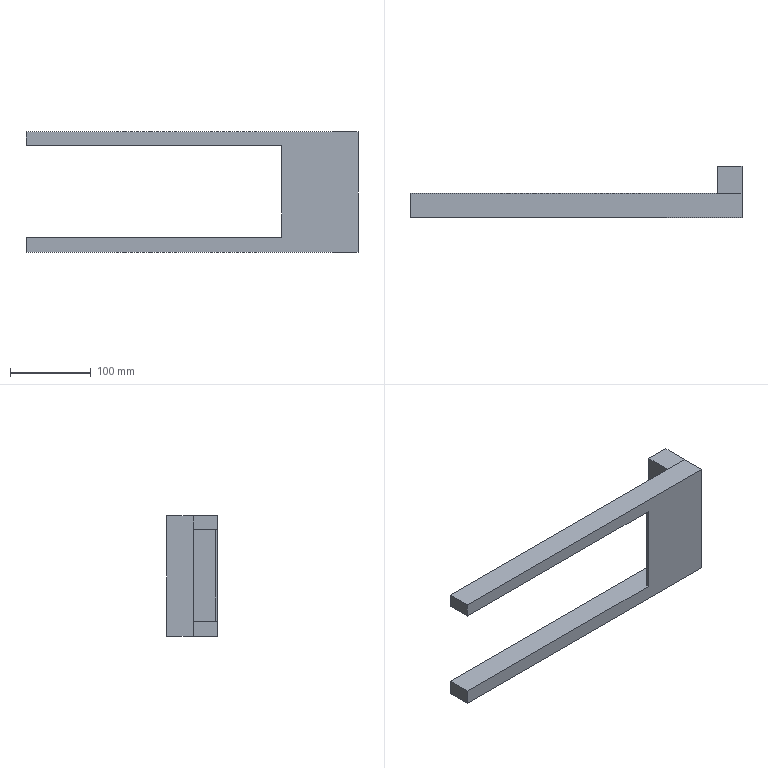Component | SolidWorks | w-1 | 2 solids | 18 faces | box 412.36 x 63.27 x 149.69 mm | volume 706312 mm3 | plane 18
STEP:
#1=CARTESIAN_POINT('',(5.039,-6.626,-2.108));
#2=VERTEX_POINT('',#1);
#3=CARTESIAN_POINT('',(5.039,-6.626,-2.842));
#4=VERTEX_POINT('',#3);
#5=CARTESIAN_POINT('',(5.039,-6.626,3.051));
#6=DIRECTION('',(0.,0.,-1.));
#7=VECTOR('',#6,39.37);
#8=LINE('',#5,#7);
#9=EDGE_CURVE('',#2,#4,#8,.T.);
#10=ORIENTED_EDGE('',*,*,#9,.F.);
#11=CARTESIAN_POINT('',(5.039,-5.445,-2.108));
#12=VERTEX_POINT('',#11);
#13=CARTESIAN_POINT('',(5.039,-8.83,-2.108));
#14=DIRECTION('',(0.,1.,0.));
#15=VECTOR('',#14,39.37);
#16=LINE('',#13,#15);
#17=EDGE_CURVE('',#2,#12,#16,.T.);
#18=ORIENTED_EDGE('',*,*,#17,.T.);
#19=CARTESIAN_POINT('',(5.039,-5.445,-2.842));
#20=VERTEX_POINT('',#19);
#21=CARTESIAN_POINT('',(5.039,-5.445,3.051));
#22=DIRECTION('',(0.,0.,-1.));
#23=VECTOR('',#22,39.37);
#24=LINE('',#21,#23);
#25=EDGE_CURVE('',#12,#20,#24,.T.);
#26=ORIENTED_EDGE('',*,*,#25,.T.);
#27=CARTESIAN_POINT('',(5.039,-6.626,-2.842));
#28=DIRECTION('',(0.,1.,0.));
#29=VECTOR('',#28,39.37);
#30=LINE('',#27,#29);
#31=EDGE_CURVE('',#4,#20,#30,.T.);
#32=ORIENTED_EDGE('',*,*,#31,.F.);
#33=EDGE_LOOP('',(#10,#18,#26,#32));
#34=FACE_OUTER_BOUND('',#33,.T.);
#35=CARTESIAN_POINT('',(5.039,-6.626,3.051));
#36=DIRECTION('',(1.,0.,0.));
#37=DIRECTION('',(0.,-1.,0.));
#38=AXIS2_PLACEMENT_3D('',#35,#36,#37);
#39=PLANE('',#38);
#40=ADVANCED_FACE('',(#34),#39,.F.);
#41=CARTESIAN_POINT('',(5.039,-5.445,3.051));
#42=VERTEX_POINT('',#41);
#43=CARTESIAN_POINT('',(5.039,-5.445,2.387));
#44=VERTEX_POINT('',#43);
#45=CARTESIAN_POINT('',(5.039,-5.445,3.051));
#46=DIRECTION('',(0.,0.,-1.));
#47=VECTOR('',#46,39.37);
#48=LINE('',#45,#47);
#49=EDGE_CURVE('',#42,#44,#48,.T.);
#50=ORIENTED_EDGE('',*,*,#49,.T.);
#51=CARTESIAN_POINT('',(5.039,-6.626,2.387));
#52=VERTEX_POINT('',#51);
#53=CARTESIAN_POINT('',(5.039,-8.83,2.387));
#54=DIRECTION('',(0.,1.,0.));
#55=VECTOR('',#54,39.37);
#56=LINE('',#53,#55);
#57=EDGE_CURVE('',#52,#44,#56,.T.);
#58=ORIENTED_EDGE('',*,*,#57,.F.);
#59=CARTESIAN_POINT('',(5.039,-6.626,3.051));
#60=VERTEX_POINT('',#59);
#61=CARTESIAN_POINT('',(5.039,-6.626,3.051));
#62=DIRECTION('',(0.,0.,-1.));
#63=VECTOR('',#62,39.37);
#64=LINE('',#61,#63);
#65=EDGE_CURVE('',#60,#52,#64,.T.);
#66=ORIENTED_EDGE('',*,*,#65,.F.);
#67=CARTESIAN_POINT('',(5.039,-6.626,3.051));
#68=DIRECTION('',(0.,1.,0.));
#69=VECTOR('',#68,39.37);
#70=LINE('',#67,#69);
#71=EDGE_CURVE('',#60,#42,#70,.T.);
#72=ORIENTED_EDGE('',*,*,#71,.T.);
#73=EDGE_LOOP('',(#50,#58,#66,#72));
#74=FACE_OUTER_BOUND('',#73,.T.);
#75=CARTESIAN_POINT('',(5.039,-6.626,3.051));
#76=DIRECTION('',(1.,0.,0.));
#77=DIRECTION('',(0.,-1.,0.));
#78=AXIS2_PLACEMENT_3D('',#75,#76,#77);
#79=PLANE('',#78);
#80=ADVANCED_FACE('',(#74),#79,.F.);
#81=CARTESIAN_POINT('',(21.274,-5.445,-2.842));
#82=VERTEX_POINT('',#81);
#83=CARTESIAN_POINT('',(5.039,-5.445,-2.842));
#84=DIRECTION('',(1.,0.,0.));
#85=VECTOR('',#84,39.37);
#86=LINE('',#83,#85);
#87=EDGE_CURVE('',#20,#82,#86,.T.);
#88=ORIENTED_EDGE('',*,*,#87,.T.);
#89=CARTESIAN_POINT('',(21.274,-6.626,-2.842));
#90=VERTEX_POINT('',#89);
#91=CARTESIAN_POINT('',(21.274,-6.626,-2.842));
#92=DIRECTION('',(0.,1.,0.));
#93=VECTOR('',#92,39.37);
#94=LINE('',#91,#93);
#95=EDGE_CURVE('',#90,#82,#94,.T.);
#96=ORIENTED_EDGE('',*,*,#95,.F.);
#97=CARTESIAN_POINT('',(5.039,-6.626,-2.842));
#98=DIRECTION('',(1.,0.,0.));
#99=VECTOR('',#98,39.37);
#100=LINE('',#97,#99);
#101=EDGE_CURVE('',#4,#90,#100,.T.);
#102=ORIENTED_EDGE('',*,*,#101,.F.);
#103=ORIENTED_EDGE('',*,*,#31,.T.);
#104=EDGE_LOOP('',(#88,#96,#102,#103));
#105=FACE_OUTER_BOUND('',#104,.T.);
#106=CARTESIAN_POINT('',(5.039,-6.626,-2.842));
#107=DIRECTION('',(-0.,0.,1.));
#108=DIRECTION('',(-1.,0.,-0.));
#109=AXIS2_PLACEMENT_3D('',#106,#107,#108);
#110=PLANE('',#109);
#111=ADVANCED_FACE('',(#105),#110,.F.);
#112=CARTESIAN_POINT('',(21.274,-5.445,3.051));
#113=VERTEX_POINT('',#112);
#114=CARTESIAN_POINT('',(21.274,-5.445,3.051));
#115=DIRECTION('',(0.,0.,1.));
#116=VECTOR('',#115,39.37);
#117=LINE('',#114,#116);
#118=EDGE_CURVE('',#82,#113,#117,.T.);
#119=ORIENTED_EDGE('',*,*,#118,.T.);
#120=CARTESIAN_POINT('',(21.274,-6.626,3.051));
#121=VERTEX_POINT('',#120);
#122=CARTESIAN_POINT('',(21.274,-6.626,3.051));
#123=DIRECTION('',(0.,1.,0.));
#124=VECTOR('',#123,39.37);
#125=LINE('',#122,#124);
#126=EDGE_CURVE('',#121,#113,#125,.T.);
#127=ORIENTED_EDGE('',*,*,#126,.F.);
#128=CARTESIAN_POINT('',(21.274,-6.626,3.051));
#129=DIRECTION('',(0.,0.,1.));
#130=VECTOR('',#129,39.37);
#131=LINE('',#128,#130);
#132=EDGE_CURVE('',#90,#121,#131,.T.);
#133=ORIENTED_EDGE('',*,*,#132,.F.);
#134=ORIENTED_EDGE('',*,*,#95,.T.);
#135=EDGE_LOOP('',(#119,#127,#133,#134));
#136=FACE_OUTER_BOUND('',#135,.T.);
#137=CARTESIAN_POINT('',(21.274,-6.626,3.051));
#138=DIRECTION('',(-1.,0.,0.));
#139=DIRECTION('',(0.,1.,0.));
#140=AXIS2_PLACEMENT_3D('',#137,#138,#139);
#141=PLANE('',#140);
#142=ADVANCED_FACE('',(#136),#141,.F.);
#143=CARTESIAN_POINT('',(5.039,-5.445,3.051));
#144=DIRECTION('',(-1.,0.,0.));
#145=VECTOR('',#144,39.37);
#146=LINE('',#143,#145);
#147=EDGE_CURVE('',#113,#42,#146,.T.);
#148=ORIENTED_EDGE('',*,*,#147,.T.);
#149=ORIENTED_EDGE('',*,*,#71,.F.);
#150=CARTESIAN_POINT('',(5.039,-6.626,3.051));
#151=DIRECTION('',(-1.,0.,0.));
#152=VECTOR('',#151,39.37);
#153=LINE('',#150,#152);
#154=EDGE_CURVE('',#121,#60,#153,.T.);
#155=ORIENTED_EDGE('',*,*,#154,.F.);
#156=ORIENTED_EDGE('',*,*,#126,.T.);
#157=EDGE_LOOP('',(#148,#149,#155,#156));
#158=FACE_OUTER_BOUND('',#157,.T.);
#159=CARTESIAN_POINT('',(5.039,-6.626,3.051));
#160=DIRECTION('',(0.,0.,-1.));
#161=DIRECTION('',(0.,-1.,0.));
#162=AXIS2_PLACEMENT_3D('',#159,#160,#161);
#163=PLANE('',#162);
#164=ADVANCED_FACE('',(#158),#163,.F.);
#165=CARTESIAN_POINT('',(17.554,-6.626,-2.108));
#166=VERTEX_POINT('',#165);
#167=CARTESIAN_POINT('',(0.,-6.626,-2.108));
#168=DIRECTION('',(1.,0.,0.));
#169=VECTOR('',#168,39.37);
#170=LINE('',#167,#169);
#171=EDGE_CURVE('',#2,#166,#170,.T.);
#172=ORIENTED_EDGE('',*,*,#171,.F.);
#173=ORIENTED_EDGE('',*,*,#9,.T.);
#174=ORIENTED_EDGE('',*,*,#101,.T.);
#175=ORIENTED_EDGE('',*,*,#132,.T.);
#176=ORIENTED_EDGE('',*,*,#154,.T.);
#177=ORIENTED_EDGE('',*,*,#65,.T.);
#178=CARTESIAN_POINT('',(17.554,-6.626,2.387));
#179=VERTEX_POINT('',#178);
#180=CARTESIAN_POINT('',(0.,-6.626,2.387));
#181=DIRECTION('',(-1.,0.,0.));
#182=VECTOR('',#181,39.37);
#183=LINE('',#180,#182);
#184=EDGE_CURVE('',#179,#52,#183,.T.);
#185=ORIENTED_EDGE('',*,*,#184,.F.);
#186=CARTESIAN_POINT('',(17.554,-6.626,-2.108));
#187=DIRECTION('',(0.,0.,-1.));
#188=VECTOR('',#187,39.37);
#189=LINE('',#186,#188);
#190=EDGE_CURVE('',#179,#166,#189,.T.);
#191=ORIENTED_EDGE('',*,*,#190,.T.);
#192=EDGE_LOOP('',(#172,#173,#174,#175,#176,#177,#185,#191));
#193=FACE_OUTER_BOUND('',#192,.T.);
#194=CARTESIAN_POINT('',(0.,-6.626,0.));
#195=DIRECTION('',(0.,-1.,0.));
#196=DIRECTION('',(-1.,0.,0.));
#197=AXIS2_PLACEMENT_3D('',#194,#195,#196);
#198=PLANE('',#197);
#199=ADVANCED_FACE('',(#193),#198,.T.);
#200=ORIENTED_EDGE('',*,*,#25,.F.);
#201=CARTESIAN_POINT('',(20.093,-5.445,-2.108));
#202=VERTEX_POINT('',#201);
#203=CARTESIAN_POINT('',(5.039,-5.445,-2.108));
#204=DIRECTION('',(-1.,0.,0.));
#205=VECTOR('',#204,39.37);
#206=LINE('',#203,#205);
#207=EDGE_CURVE('',#202,#12,#206,.T.);
#208=ORIENTED_EDGE('',*,*,#207,.F.);
#209=CARTESIAN_POINT('',(20.093,-5.445,2.387));
#210=VERTEX_POINT('',#209);
#211=CARTESIAN_POINT('',(20.093,-5.445,-2.108));
#212=DIRECTION('',(0.,0.,-1.));
#213=VECTOR('',#212,39.37);
#214=LINE('',#211,#213);
#215=EDGE_CURVE('',#210,#202,#214,.T.);
#216=ORIENTED_EDGE('',*,*,#215,.F.);
#217=CARTESIAN_POINT('',(5.039,-5.445,2.387));
#218=DIRECTION('',(1.,0.,0.));
#219=VECTOR('',#218,39.37);
#220=LINE('',#217,#219);
#221=EDGE_CURVE('',#44,#210,#220,.T.);
#222=ORIENTED_EDGE('',*,*,#221,.F.);
#223=ORIENTED_EDGE('',*,*,#49,.F.);
#224=ORIENTED_EDGE('',*,*,#147,.F.);
#225=ORIENTED_EDGE('',*,*,#118,.F.);
#226=ORIENTED_EDGE('',*,*,#87,.F.);
#227=EDGE_LOOP('',(#200,#208,#216,#222,#223,#224,#225,#226));
#228=FACE_OUTER_BOUND('',#227,.T.);
#229=CARTESIAN_POINT('',(0.,-5.445,0.));
#230=DIRECTION('',(0.,-1.,0.));
#231=DIRECTION('',(-1.,0.,0.));
#232=AXIS2_PLACEMENT_3D('',#229,#230,#231);
#233=PLANE('',#232);
#234=ADVANCED_FACE('',(#228),#233,.F.);
#235=ORIENTED_EDGE('',*,*,#171,.T.);
#236=CARTESIAN_POINT('',(17.554,-6.547,-2.108));
#237=VERTEX_POINT('',#236);
#238=CARTESIAN_POINT('',(17.554,-6.547,-2.108));
#239=DIRECTION('',(0.,-1.,0.));
#240=VECTOR('',#239,39.37);
#241=LINE('',#238,#240);
#242=EDGE_CURVE('',#237,#166,#241,.T.);
#243=ORIENTED_EDGE('',*,*,#242,.F.);
#244=CARTESIAN_POINT('',(20.093,-6.547,-2.108));
#245=VERTEX_POINT('',#244);
#246=CARTESIAN_POINT('',(17.554,-6.547,-2.108));
#247=DIRECTION('',(1.,0.,0.));
#248=VECTOR('',#247,39.37);
#249=LINE('',#246,#248);
#250=EDGE_CURVE('',#237,#245,#249,.T.);
#251=ORIENTED_EDGE('',*,*,#250,.T.);
#252=CARTESIAN_POINT('',(20.093,-8.83,-2.108));
#253=DIRECTION('',(0.,1.,0.));
#254=VECTOR('',#253,39.37);
#255=LINE('',#252,#254);
#256=EDGE_CURVE('',#245,#202,#255,.T.);
#257=ORIENTED_EDGE('',*,*,#256,.T.);
#258=ORIENTED_EDGE('',*,*,#207,.T.);
#259=ORIENTED_EDGE('',*,*,#17,.F.);
#260=EDGE_LOOP('',(#235,#243,#251,#257,#258,#259));
#261=FACE_OUTER_BOUND('',#260,.T.);
#262=CARTESIAN_POINT('',(5.039,-8.83,-2.108));
#263=DIRECTION('',(0.,0.,-1.));
#264=DIRECTION('',(0.,-1.,0.));
#265=AXIS2_PLACEMENT_3D('',#262,#263,#264);
#266=PLANE('',#265);
#267=ADVANCED_FACE('',(#261),#266,.F.);
#268=ORIENTED_EDGE('',*,*,#256,.F.);
#269=CARTESIAN_POINT('',(20.093,-6.547,2.387));
#270=VERTEX_POINT('',#269);
#271=CARTESIAN_POINT('',(20.093,-6.547,-2.108));
#272=DIRECTION('',(0.,0.,1.));
#273=VECTOR('',#272,39.37);
#274=LINE('',#271,#273);
#275=EDGE_CURVE('',#245,#270,#274,.T.);
#276=ORIENTED_EDGE('',*,*,#275,.T.);
#277=CARTESIAN_POINT('',(20.093,-8.83,2.387));
#278=DIRECTION('',(0.,1.,0.));
#279=VECTOR('',#278,39.37);
#280=LINE('',#277,#279);
#281=EDGE_CURVE('',#270,#210,#280,.T.);
#282=ORIENTED_EDGE('',*,*,#281,.T.);
#283=ORIENTED_EDGE('',*,*,#215,.T.);
#284=EDGE_LOOP('',(#268,#276,#282,#283));
#285=FACE_OUTER_BOUND('',#284,.T.);
#286=CARTESIAN_POINT('',(20.093,-8.83,-2.108));
#287=DIRECTION('',(1.,0.,0.));
#288=DIRECTION('',(0.,-1.,0.));
#289=AXIS2_PLACEMENT_3D('',#286,#287,#288);
#290=PLANE('',#289);
#291=ADVANCED_FACE('',(#285),#290,.F.);
#292=CARTESIAN_POINT('',(17.554,-6.547,2.387));
#293=VERTEX_POINT('',#292);
#294=CARTESIAN_POINT('',(17.554,-6.547,2.387));
#295=DIRECTION('',(-1.,0.,0.));
#296=VECTOR('',#295,39.37);
#297=LINE('',#294,#296);
#298=EDGE_CURVE('',#270,#293,#297,.T.);
#299=ORIENTED_EDGE('',*,*,#298,.T.);
#300=CARTESIAN_POINT('',(17.554,-6.547,2.387));
#301=DIRECTION('',(0.,-1.,0.));
#302=VECTOR('',#301,39.37);
#303=LINE('',#300,#302);
#304=EDGE_CURVE('',#293,#179,#303,.T.);
#305=ORIENTED_EDGE('',*,*,#304,.T.);
#306=ORIENTED_EDGE('',*,*,#184,.T.);
#307=ORIENTED_EDGE('',*,*,#57,.T.);
#308=ORIENTED_EDGE('',*,*,#221,.T.);
#309=ORIENTED_EDGE('',*,*,#281,.F.);
#310=EDGE_LOOP('',(#299,#305,#306,#307,#308,#309));
#311=FACE_OUTER_BOUND('',#310,.T.);
#312=CARTESIAN_POINT('',(5.039,-8.83,2.387));
#313=DIRECTION('',(0.,0.,1.));
#314=DIRECTION('',(0.,1.,0.));
#315=AXIS2_PLACEMENT_3D('',#312,#313,#314);
#316=PLANE('',#315);
#317=ADVANCED_FACE('',(#311),#316,.F.);
#318=ORIENTED_EDGE('',*,*,#190,.F.);
#319=ORIENTED_EDGE('',*,*,#304,.F.);
#320=CARTESIAN_POINT('',(17.554,-6.547,-2.108));
#321=DIRECTION('',(0.,0.,-1.));
#322=VECTOR('',#321,39.37);
#323=LINE('',#320,#322);
#324=EDGE_CURVE('',#293,#237,#323,.T.);
#325=ORIENTED_EDGE('',*,*,#324,.T.);
#326=ORIENTED_EDGE('',*,*,#242,.T.);
#327=EDGE_LOOP('',(#318,#319,#325,#326));
#328=FACE_OUTER_BOUND('',#327,.T.);
#329=CARTESIAN_POINT('',(17.554,-6.547,-2.108));
#330=DIRECTION('',(-1.,0.,0.));
#331=DIRECTION('',(0.,1.,0.));
#332=AXIS2_PLACEMENT_3D('',#329,#330,#331);
#333=PLANE('',#332);
#334=ADVANCED_FACE('',(#328),#333,.T.);
#335=ORIENTED_EDGE('',*,*,#324,.F.);
#336=ORIENTED_EDGE('',*,*,#298,.F.);
#337=ORIENTED_EDGE('',*,*,#275,.F.);
#338=ORIENTED_EDGE('',*,*,#250,.F.);
#339=EDGE_LOOP('',(#335,#336,#337,#338));
#340=FACE_OUTER_BOUND('',#339,.T.);
#341=CARTESIAN_POINT('',(0.,-6.547,0.));
#342=DIRECTION('',(0.,1.,0.));
#343=DIRECTION('',(1.,0.,0.));
#344=AXIS2_PLACEMENT_3D('',#341,#342,#343);
#345=PLANE('',#344);
#346=ADVANCED_FACE('',(#340),#345,.T.);
#347=CLOSED_SHELL('',(#40,#80,#111,#142,#164,#199,#234,#267,#291,#317,#334,#346));
#348=MANIFOLD_SOLID_BREP('',#347);
#349=CARTESIAN_POINT('',(21.274,-5.445,3.051));
#350=VERTEX_POINT('',#349);
#351=CARTESIAN_POINT('',(21.274,-5.445,-2.842));
#352=VERTEX_POINT('',#351);
#353=CARTESIAN_POINT('',(21.274,-5.445,3.051));
#354=DIRECTION('',(0.,0.,-1.));
#355=VECTOR('',#354,39.37);
#356=LINE('',#353,#355);
#357=EDGE_CURVE('',#350,#352,#356,.T.);
#358=ORIENTED_EDGE('',*,*,#357,.F.);
#359=CARTESIAN_POINT('',(20.093,-5.445,3.051));
#360=VERTEX_POINT('',#359);
#361=CARTESIAN_POINT('',(20.093,-5.445,3.051));
#362=DIRECTION('',(1.,0.,0.));
#363=VECTOR('',#362,39.37);
#364=LINE('',#361,#363);
#365=EDGE_CURVE('',#360,#350,#364,.T.);
#366=ORIENTED_EDGE('',*,*,#365,.F.);
#367=CARTESIAN_POINT('',(20.093,-5.445,-2.842));
#368=VERTEX_POINT('',#367);
#369=CARTESIAN_POINT('',(20.093,-5.445,3.051));
#370=DIRECTION('',(0.,0.,-1.));
#371=VECTOR('',#370,39.37);
#372=LINE('',#369,#371);
#373=EDGE_CURVE('',#360,#368,#372,.T.);
#374=ORIENTED_EDGE('',*,*,#373,.T.);
#375=CARTESIAN_POINT('',(20.093,-5.445,-2.842));
#376=DIRECTION('',(1.,0.,0.));
#377=VECTOR('',#376,39.37);
#378=LINE('',#375,#377);
#379=EDGE_CURVE('',#368,#352,#378,.T.);
#380=ORIENTED_EDGE('',*,*,#379,.T.);
#381=EDGE_LOOP('',(#358,#366,#374,#380));
#382=FACE_OUTER_BOUND('',#381,.T.);
#383=CARTESIAN_POINT('',(20.093,-5.445,3.051));
#384=DIRECTION('',(0.,-1.,0.));
#385=DIRECTION('',(-1.,0.,0.));
#386=AXIS2_PLACEMENT_3D('',#383,#384,#385);
#387=PLANE('',#386);
#388=ADVANCED_FACE('',(#382),#387,.T.);
#389=CARTESIAN_POINT('',(21.274,-4.135,3.051));
#390=VERTEX_POINT('',#389);
#391=CARTESIAN_POINT('',(21.274,-5.445,3.051));
#392=DIRECTION('',(0.,-1.,0.));
#393=VECTOR('',#392,39.37);
#394=LINE('',#391,#393);
#395=EDGE_CURVE('',#390,#350,#394,.T.);
#396=ORIENTED_EDGE('',*,*,#395,.F.);
#397=CARTESIAN_POINT('',(20.093,-4.135,3.051));
#398=VERTEX_POINT('',#397);
#399=CARTESIAN_POINT('',(20.093,-4.135,3.051));
#400=DIRECTION('',(1.,0.,0.));
#401=VECTOR('',#400,39.37);
#402=LINE('',#399,#401);
#403=EDGE_CURVE('',#398,#390,#402,.T.);
#404=ORIENTED_EDGE('',*,*,#403,.F.);
#405=CARTESIAN_POINT('',(20.093,-5.445,3.051));
#406=DIRECTION('',(0.,-1.,0.));
#407=VECTOR('',#406,39.37);
#408=LINE('',#405,#407);
#409=EDGE_CURVE('',#398,#360,#408,.T.);
#410=ORIENTED_EDGE('',*,*,#409,.T.);
#411=ORIENTED_EDGE('',*,*,#365,.T.);
#412=EDGE_LOOP('',(#396,#404,#410,#411));
#413=FACE_OUTER_BOUND('',#412,.T.);
#414=CARTESIAN_POINT('',(20.093,-5.445,3.051));
#415=DIRECTION('',(0.,0.,1.));
#416=DIRECTION('',(0.,1.,0.));
#417=AXIS2_PLACEMENT_3D('',#414,#415,#416);
#418=PLANE('',#417);
#419=ADVANCED_FACE('',(#413),#418,.T.);
#420=CARTESIAN_POINT('',(21.274,-4.135,-2.842));
#421=VERTEX_POINT('',#420);
#422=CARTESIAN_POINT('',(21.274,-4.135,3.051));
#423=DIRECTION('',(0.,0.,1.));
#424=VECTOR('',#423,39.37);
#425=LINE('',#422,#424);
#426=EDGE_CURVE('',#421,#390,#425,.T.);
#427=ORIENTED_EDGE('',*,*,#426,.F.);
#428=CARTESIAN_POINT('',(20.093,-4.135,-2.842));
#429=VERTEX_POINT('',#428);
#430=CARTESIAN_POINT('',(20.093,-4.135,-2.842));
#431=DIRECTION('',(1.,0.,0.));
#432=VECTOR('',#431,39.37);
#433=LINE('',#430,#432);
#434=EDGE_CURVE('',#429,#421,#433,.T.);
#435=ORIENTED_EDGE('',*,*,#434,.F.);
#436=CARTESIAN_POINT('',(20.093,-4.135,3.051));
#437=DIRECTION('',(0.,0.,1.));
#438=VECTOR('',#437,39.37);
#439=LINE('',#436,#438);
#440=EDGE_CURVE('',#429,#398,#439,.T.);
#441=ORIENTED_EDGE('',*,*,#440,.T.);
#442=ORIENTED_EDGE('',*,*,#403,.T.);
#443=EDGE_LOOP('',(#427,#435,#441,#442));
#444=FACE_OUTER_BOUND('',#443,.T.);
#445=CARTESIAN_POINT('',(20.093,-4.135,3.051));
#446=DIRECTION('',(0.,1.,0.));
#447=DIRECTION('',(1.,0.,0.));
#448=AXIS2_PLACEMENT_3D('',#445,#446,#447);
#449=PLANE('',#448);
#450=ADVANCED_FACE('',(#444),#449,.T.);
#451=CARTESIAN_POINT('',(21.274,-5.445,-2.842));
#452=DIRECTION('',(0.,1.,0.));
#453=VECTOR('',#452,39.37);
#454=LINE('',#451,#453);
#455=EDGE_CURVE('',#352,#421,#454,.T.);
#456=ORIENTED_EDGE('',*,*,#455,.F.);
#457=ORIENTED_EDGE('',*,*,#379,.F.);
#458=CARTESIAN_POINT('',(20.093,-5.445,-2.842));
#459=DIRECTION('',(0.,1.,0.));
#460=VECTOR('',#459,39.37);
#461=LINE('',#458,#460);
#462=EDGE_CURVE('',#368,#429,#461,.T.);
#463=ORIENTED_EDGE('',*,*,#462,.T.);
#464=ORIENTED_EDGE('',*,*,#434,.T.);
#465=EDGE_LOOP('',(#456,#457,#463,#464));
#466=FACE_OUTER_BOUND('',#465,.T.);
#467=CARTESIAN_POINT('',(20.093,-5.445,-2.842));
#468=DIRECTION('',(0.,0.,-1.));
#469=DIRECTION('',(0.,-1.,0.));
#470=AXIS2_PLACEMENT_3D('',#467,#468,#469);
#471=PLANE('',#470);
#472=ADVANCED_FACE('',(#466),#471,.T.);
#473=ORIENTED_EDGE('',*,*,#373,.F.);
#474=ORIENTED_EDGE('',*,*,#409,.F.);
#475=ORIENTED_EDGE('',*,*,#440,.F.);
#476=ORIENTED_EDGE('',*,*,#462,.F.);
#477=EDGE_LOOP('',(#473,#474,#475,#476));
#478=FACE_OUTER_BOUND('',#477,.T.);
#479=CARTESIAN_POINT('',(20.093,-5.445,0.));
#480=DIRECTION('',(1.,0.,0.));
#481=DIRECTION('',(0.,-1.,0.));
#482=AXIS2_PLACEMENT_3D('',#479,#480,#481);
#483=PLANE('',#482);
#484=ADVANCED_FACE('',(#478),#483,.F.);
#485=ORIENTED_EDGE('',*,*,#357,.T.);
#486=ORIENTED_EDGE('',*,*,#455,.T.);
#487=ORIENTED_EDGE('',*,*,#426,.T.);
#488=ORIENTED_EDGE('',*,*,#395,.T.);
#489=EDGE_LOOP('',(#485,#486,#487,#488));
#490=FACE_OUTER_BOUND('',#489,.T.);
#491=CARTESIAN_POINT('',(21.274,-5.445,0.));
#492=DIRECTION('',(1.,0.,0.));
#493=DIRECTION('',(0.,-1.,0.));
#494=AXIS2_PLACEMENT_3D('',#491,#492,#493);
#495=PLANE('',#494);
#496=ADVANCED_FACE('',(#490),#495,.T.);
#497=CLOSED_SHELL('',(#388,#419,#450,#472,#484,#496));
#498=MANIFOLD_SOLID_BREP('',#497);
#499=CARTESIAN_POINT('',(0.,0.,0.));
#500=DIRECTION('',(0.,0.,1.));
#501=DIRECTION('',(1.,0.,0.));
#502=AXIS2_PLACEMENT_3D('',#499,#500,#501);
#503=(LENGTH_UNIT()NAMED_UNIT(*)SI_UNIT($,.METRE.));
#504=LENGTH_MEASURE_WITH_UNIT(LENGTH_MEASURE(0.0254),#503);
#505=DIMENSIONAL_EXPONENTS(1.,0.,0.,0.,0.,0.,0.);
#506=(CONVERSION_BASED_UNIT('',#504)LENGTH_UNIT()NAMED_UNIT(#505));
#507=UNCERTAINTY_MEASURE_WITH_UNIT(LENGTH_MEASURE(0.00001),#506,'','');
#508=(NAMED_UNIT(*)PLANE_ANGLE_UNIT()SI_UNIT($,.RADIAN.));
#509=(NAMED_UNIT(*)SI_UNIT($,.STERADIAN.)SOLID_ANGLE_UNIT());
#510=(GEOMETRIC_REPRESENTATION_CONTEXT(3)GLOBAL_UNCERTAINTY_ASSIGNED_CONTEXT((#507))GLOBAL_UNIT_ASSIGNED_CONTEXT((#506,#508,#509))REPRESENTATION_CONTEXT('',''));
#511=ADVANCED_BREP_SHAPE_REPRESENTATION('',(#348,#498,#502),#510);
#512=COLOUR_RGB('',0.7922,0.8196,0.9333);
#513=FILL_AREA_STYLE_COLOUR('',#512);
#514=FILL_AREA_STYLE('',(#513));
#515=SURFACE_STYLE_FILL_AREA(#514);
#516=SURFACE_SIDE_STYLE('',(#515));
#517=SURFACE_STYLE_USAGE(.BOTH.,#516);
#518=PRESENTATION_STYLE_ASSIGNMENT((#517));
#519=STYLED_ITEM('',(#518),#498);
#520=PRESENTATION_LAYER_ASSIGNMENT('','',(#519));
#521=(LENGTH_UNIT()NAMED_UNIT(*)SI_UNIT($,.METRE.));
#522=LENGTH_MEASURE_WITH_UNIT(LENGTH_MEASURE(0.0254),#521);
#523=DIMENSIONAL_EXPONENTS(1.,0.,0.,0.,0.,0.,0.);
#524=(CONVERSION_BASED_UNIT('',#522)LENGTH_UNIT()NAMED_UNIT(#523));
#525=UNCERTAINTY_MEASURE_WITH_UNIT(LENGTH_MEASURE(0.00001),#524,'','');
#526=(NAMED_UNIT(*)PLANE_ANGLE_UNIT()SI_UNIT($,.RADIAN.));
#527=(NAMED_UNIT(*)SI_UNIT($,.STERADIAN.)SOLID_ANGLE_UNIT());
#528=(GEOMETRIC_REPRESENTATION_CONTEXT(3)GLOBAL_UNCERTAINTY_ASSIGNED_CONTEXT((#525))GLOBAL_UNIT_ASSIGNED_CONTEXT((#524,#526,#527))REPRESENTATION_CONTEXT('',''));
#529=MECHANICAL_DESIGN_GEOMETRIC_PRESENTATION_REPRESENTATION('',(#519),#528);
#530=COLOUR_RGB('',0.7922,0.8196,0.9333);
#531=FILL_AREA_STYLE_COLOUR('',#530);
#532=FILL_AREA_STYLE('',(#531));
#533=SURFACE_STYLE_FILL_AREA(#532);
#534=SURFACE_SIDE_STYLE('',(#533));
#535=SURFACE_STYLE_USAGE(.BOTH.,#534);
#536=PRESENTATION_STYLE_ASSIGNMENT((#535));
#537=STYLED_ITEM('',(#536),#348);
#538=(LENGTH_UNIT()NAMED_UNIT(*)SI_UNIT($,.METRE.));
#539=LENGTH_MEASURE_WITH_UNIT(LENGTH_MEASURE(0.0254),#538);
#540=DIMENSIONAL_EXPONENTS(1.,0.,0.,0.,0.,0.,0.);
#541=(CONVERSION_BASED_UNIT('',#539)LENGTH_UNIT()NAMED_UNIT(#540));
#542=UNCERTAINTY_MEASURE_WITH_UNIT(LENGTH_MEASURE(0.00001),#541,'','');
#543=(NAMED_UNIT(*)PLANE_ANGLE_UNIT()SI_UNIT($,.RADIAN.));
#544=(NAMED_UNIT(*)SI_UNIT($,.STERADIAN.)SOLID_ANGLE_UNIT());
#545=(GEOMETRIC_REPRESENTATION_CONTEXT(3)GLOBAL_UNCERTAINTY_ASSIGNED_CONTEXT((#542))GLOBAL_UNIT_ASSIGNED_CONTEXT((#541,#543,#544))REPRESENTATION_CONTEXT('',''));
#546=MECHANICAL_DESIGN_GEOMETRIC_PRESENTATION_REPRESENTATION('',(#537),#545);
#547=PRESENTATION_LAYER_ASSIGNMENT('','',(#537));